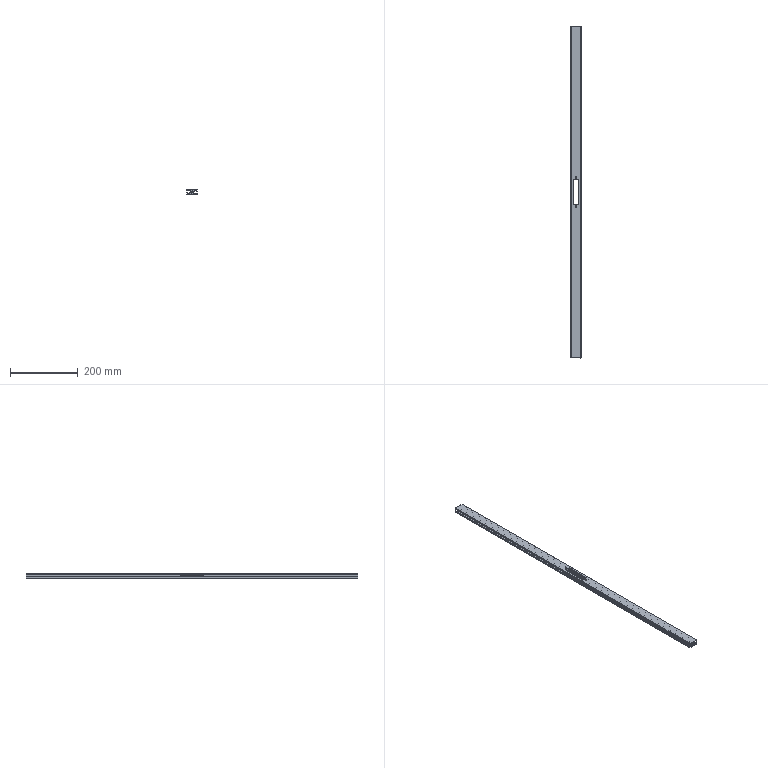Component | SolidWorks | 2012MB0201-1_ASideDoor-1-1_A3005-1 | 1 solid | 68 faces | box 30.3 x 982 x 15.67 mm | volume 226049 mm3 | plane 48 | cylinder 20 | commonest cylinder face diameters 4.5 x8 6 x4 5 x4 2 x4
build123d program:
from build123d import *

# Parameters (mm, degrees)
SKETCH1_2_W                 = 30
SKETCH1_2_H                 = 15
BOSS_EXTRUDE1_DEPTH         = 982
SKETCH2_2_R                 = 2.5
CUT_EXTRUDE1_DEPTH          = 983.143
FILLET1_R                   = 1
SKETCH1_3_R                 = 2.25
SKETCH1_3_W                 = 16.5
SKETCH1_3_H                 = 73
CUT_EXTRUDE1_2_DEPTH        = 983.229
SKETCH1_R                   = 3
M6_THREADED_END_HOLE1_DEPTH = 13
M6_START                    = -13
SKETCH2_R                   = 3
M6_THREADED_END_HOLE2_DEPTH = 13


with BuildPart() as part:
    # Sketch1_2 → Boss-Extrude1 (new body)
    with BuildSketch(Plane(origin=(0, 0, 0), x_dir=(1, 0, 0), z_dir=(0, 1, 0))):
        Rectangle(SKETCH1_2_W, SKETCH1_2_H)
    extrude(amount=BOSS_EXTRUDE1_DEPTH)

    # Sketch2_2 → Cut-Extrude1 (cut, through all)
    with BuildSketch(Plane.XZ):
        with Locations(Location((0, 0, 0), (0, 0, 270))):
            Circle(SKETCH2_2_R)
        Polygon((15, -3.25), (12.6, -3.25), (12.6, -5.3), (6.6, -5.3), (6.6, -2.926), (4.2, -2.926), (4.2, 2.926), (6.6, 2.926), (6.6, 5.3), (12.6, 5.3), (12.6, 3.25), (15, 3.25), align=None)
        Polygon((-6.6, -2.926), (-4.2, -2.926), (-4.2, 2.926), (-6.6, 2.926), (-6.6, 5.3), (-12.6, 5.3), (-12.6, 3.25), (-15, 3.25), (-15, -3.25), (-12.6, -3.25), (-12.6, -5.3), (-6.6, -5.3), align=None)
    extrude(amount=-CUT_EXTRUDE1_DEPTH, mode=Mode.SUBTRACT)

    # Fillet1
    fillet1_edges = [part.edges().sort_by_distance(p)[0] for p in [
        (15, 491, 7.5),
        (-15, 491, 7.5),
        (-15, 491, -7.5),
        (15, 491, -7.5),
    ]]
    fillet(fillet1_edges, radius=FILLET1_R)

    # Sketch1_3 → Cut-Extrude1_2 (cut, through all)
    with BuildSketch(Plane.XY.offset(7.5)):
        with Locations((0, 533.5)):
            Circle(SKETCH1_3_R)
        with Locations((0, 448.5)):
            Circle(SKETCH1_3_R)
        with Locations((0, 491)):
            Rectangle(SKETCH1_3_W, SKETCH1_3_H)
    extrude(amount=-CUT_EXTRUDE1_2_DEPTH, mode=Mode.SUBTRACT)

    # Sketch1 → M6 Threaded End Hole1 (cut)
    with BuildSketch(Plane.XZ):
        with Locations(Location((0, 0, 0), (0, 0, 270))):
            Circle(SKETCH1_R)
    extrude(amount=-M6_THREADED_END_HOLE1_DEPTH, mode=Mode.SUBTRACT)

    # Sketch2 → M6 Threaded End Hole2 (cut)
    with BuildSketch(Plane(origin=(0, 982, 0), x_dir=(1, 0, 0), z_dir=(0, 1, 0)).offset(M6_START)):
        with Locations(Location((0, 0, 0), (0, 0, 90))):
            Circle(SKETCH2_R)
    extrude(amount=M6_THREADED_END_HOLE2_DEPTH, mode=Mode.SUBTRACT)


solid = part.part

# Placed as in the assembly
solid = solid.moved(Location((-1264.803, 972.35, -179.253), (-180, -1.371, 0)))